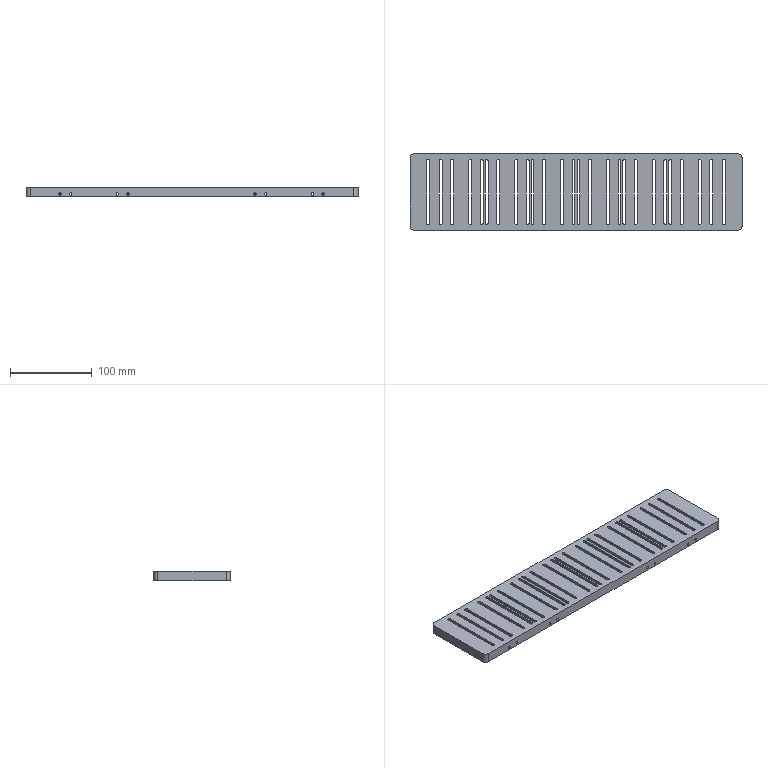Component | SolidWorks | MGL-PACK-02-00WeldedPlate2Assembly-1_MGL-PACK-02-01WeldedPlate2-1 | 1 solid | 295 faces | box 405 x 93 x 12 mm | volume 207669 mm3 | plane 151 | cylinder 92 | cone 52 | commonest cylinder face diameters 3.5 x48 3 x32 10 x8 4 x4
build123d program:
from build123d import *

# Parameters (mm, degrees)
SKETCH1_W             = 405
SKETCH1_H             = 93
BOSS_EXTRUDE1_DEPTH   = 12
CUT_EXTRUDE6_DEPTH    = 12
CUT_EXTRUDE1_DEPTH    = 12
LPATTERN1_COUNT       = 5
LPATTERN1_PITCH       = 56
CUT_EXTRUDE7_DEPTH    = 12
CUT_EXTRUDE2_DEPTH    = 6
FILLET1_R             = 5
M3_TAPPED_HOLE1_D     = 3
M3_TAPPED_HOLE1_DEPTH = 100
M3_TAPPED_HOLE1_TIP   = 0.9013
SKETCH10_W            = 9
SKETCH10_H            = 8
CUT_EXTRUDE5_DEPTH    = 2
CHAMFER2_SIZE         = 1
CHAMFER4_SIZE         = 1
CHAMFER4_SIZE2        = 3.732


with BuildPart() as part:
    # Sketch1 → Boss-Extrude1 (new body)
    with BuildSketch(Plane.XY):
        Rectangle(SKETCH1_W, SKETCH1_H)
    extrude(amount=BOSS_EXTRUDE1_DEPTH)

    # Sketch11 → Cut-Extrude6 (cut)
    with BuildSketch(Plane.XY.offset(12)):
        with BuildLine():
            Line((-178.75, 38), (-178.75, -38))
            ThreePointArc((-178.75, -38), (-180.5, -39.75), (-182.25, -38))
            Line((-182.25, -38), (-182.25, 38))
            ThreePointArc((-182.25, 38), (-180.5, 39.75), (-178.75, 38))
        make_face()
        with BuildLine():
            Line((182.25, 38), (182.25, -38))
            ThreePointArc((182.25, -38), (180.5, -39.75), (178.75, -38))
            Line((178.75, -38), (178.75, 38))
            ThreePointArc((178.75, 38), (180.5, 39.75), (182.25, 38))
        make_face()
        with BuildLine():
            Line((-163.25, 38), (-163.25, -38))
            ThreePointArc((-163.25, -38), (-165, -39.75), (-166.75, -38))
            Line((-166.75, -38), (-166.75, 38))
            ThreePointArc((-166.75, 38), (-165, 39.75), (-163.25, 38))
        make_face()
        with BuildLine():
            Line((166.75, 38), (166.75, -38))
            ThreePointArc((166.75, -38), (165, -39.75), (163.25, -38))
            Line((163.25, -38), (163.25, 38))
            ThreePointArc((163.25, 38), (165, 39.75), (166.75, 38))
        make_face()
    extrude(amount=-CUT_EXTRUDE6_DEPTH, mode=Mode.SUBTRACT)

    # Sketch2 → Cut-Extrude1 (cut)
    with BuildSketch(Plane.XY.offset(12)):
        with BuildLine():
            Line((-149.25, 38), (-149.25, -38))
            ThreePointArc((-149.25, -38), (-151, -39.75), (-152.75, -38))
            Line((-152.75, -38), (-152.75, 38))
            ThreePointArc((-152.75, 38), (-151, 39.75), (-149.25, 38))
        make_face()
        with BuildLine():
            Line((-127.25, 38), (-127.25, -38))
            ThreePointArc((-127.25, -38), (-129, -39.75), (-130.75, -38))
            Line((-130.75, -38), (-130.75, 38))
            ThreePointArc((-130.75, 38), (-129, 39.75), (-127.25, 38))
        make_face()
        with BuildLine():
            Line((-113.25, 38), (-113.25, -38))
            ThreePointArc((-113.25, -38), (-115, -39.75), (-116.75, -38))
            Line((-116.75, -38), (-116.75, 38))
            ThreePointArc((-116.75, 38), (-115, 39.75), (-113.25, 38))
        make_face()
        with BuildLine():
            Line((-107.25, 38), (-107.25, -38))
            ThreePointArc((-107.25, -38), (-109, -39.75), (-110.75, -38))
            Line((-110.75, -38), (-110.75, 38))
            ThreePointArc((-110.75, 38), (-109, 39.75), (-107.25, 38))
        make_face()
    cut_extrude1 = extrude(amount=-CUT_EXTRUDE1_DEPTH, mode=Mode.SUBTRACT)

    # LPattern1: Cut-Extrude1 ×5
    with Locations(*[(i * LPATTERN1_PITCH, 0, 0) for i in range(1, LPATTERN1_COUNT)]):
        add(cut_extrude1, mode=Mode.SUBTRACT)

    # Sketch12 → Cut-Extrude7 (cut)
    with BuildSketch(Plane.XY.offset(12)):
        with BuildLine():
            Line((131, 38), (131, -38))
            ThreePointArc((131, -38), (129, -40), (127, -38))
            Line((127, -38), (127, 38))
            ThreePointArc((127, 38), (129, 40), (131, 38))
        make_face()
        with BuildLine():
            Line((153, 38), (153, -38))
            ThreePointArc((153, -38), (151, -40), (149, -38))
            Line((149, -38), (149, 38))
            ThreePointArc((149, 38), (151, 40), (153, 38))
        make_face()
    extrude(amount=-CUT_EXTRUDE7_DEPTH, mode=Mode.SUBTRACT)

    # Sketch3 → Cut-Extrude2 (cut)
    with BuildSketch(Plane.XY.offset(12)):
        with BuildLine():
            Line((-185, 42), (185, 42))
            ThreePointArc((185, 42), (188.536, 40.536), (190, 37))
            Line((190, 37), (190, -37))
            ThreePointArc((190, -37), (188.536, -40.536), (185, -42))
            Line((185, -42), (-185, -42))
            ThreePointArc((-185, -42), (-188.536, -40.536), (-190, -37))
            Line((-190, -37), (-190, 37))
            ThreePointArc((-190, 37), (-188.536, 40.536), (-185, 42))
        make_face()
    extrude(amount=-CUT_EXTRUDE2_DEPTH, mode=Mode.SUBTRACT)

    # Fillet1
    fillet1_edges = [part.edges().sort_by_distance(p)[0] for p in [
        (-202.5, 46.5, 6),
        (202.5, 46.5, 6),
        (202.5, -46.5, 6),
        (-202.5, -46.5, 6),
    ]]
    fillet(fillet1_edges, radius=FILLET1_R)

    # M3 Tapped Hole1
    with Locations(Plane(origin=(0, -46.5, 0), x_dir=(-1, 0, 0), z_dir=(0, -1, 0))):
        with Locations((-161.05, -8.5), (-148.05, -8.5), (159.95, -8.5), (146.95, -8.5), (-91.05, -8.5), (-78.05, -8.5), (89.95, -8.5), (76.95, -8.5)):
            Hole(M3_TAPPED_HOLE1_D / 2, depth=M3_TAPPED_HOLE1_DEPTH)
            with Locations((0, 0, -(M3_TAPPED_HOLE1_DEPTH + M3_TAPPED_HOLE1_TIP / 2))):  # 118° drill point
                Cone(0, M3_TAPPED_HOLE1_D / 2, M3_TAPPED_HOLE1_TIP, mode=Mode.SUBTRACT)

    # Sketch10 → Cut-Extrude5 (cut)
    with BuildSketch(Plane.XY.offset(12)):
        with Locations((196.25, 31)):
            Rectangle(SKETCH10_W, SKETCH10_H)
        with Locations((196.25, -31)):
            Rectangle(SKETCH10_W, SKETCH10_H)
        with Locations((-196.25, 31)):
            Rectangle(SKETCH10_W, SKETCH10_H)
        with Locations((-196.25, -31)):
            Rectangle(SKETCH10_W, SKETCH10_H)
    extrude(amount=-CUT_EXTRUDE5_DEPTH, mode=Mode.SUBTRACT)

    # Chamfer2
    chamfer2_edges = [part.edges().sort_by_distance(p)[0] for p in [
        (191.75, 31, 12),
        (196.25, 27, 12),
        (200.75, 31, 12),
        (196.25, 35, 12),
        (191.75, -31, 12),
        (196.25, -35, 12),
        (200.75, -31, 12),
        (196.25, -27, 12),
        (-200.75, 31, 12),
        (-196.25, 27, 12),
        (-191.75, 31, 12),
        (-196.25, 35, 12),
        (-200.75, -31, 12),
        (-196.25, -35, 12),
        (-191.75, -31, 12),
        (-196.25, -27, 12),
    ]]
    chamfer(chamfer2_edges, length=CHAMFER2_SIZE)

    # Chamfer4
    chamfer4_edges = [part.edges().sort_by_distance(p)[0] for p in [
        (149, 0, 6),
        (153, 0, 6),
        (151, 40, 6),
        (151, -40, 6),
        (131, 0, 6),
        (129, 40, 6),
        (127, 0, 6),
        (129, -40, 6),
        (115, 39.75, 6),
        (113.25, 0, 6),
        (115, -39.75, 6),
        (116.75, 0, 6),
        (73, 39.75, 6),
        (71.25, 0, 6),
        (73, -39.75, 6),
        (74.75, 0, 6),
        (95, 39.75, 6),
        (93.25, 0, 6),
        (95, -39.75, 6),
        (96.75, 0, 6),
        (109, 39.75, 6),
        (107.25, 0, 6),
        (109, -39.75, 6),
        (110.75, 0, 6),
        (59, 39.75, 6),
        (57.25, 0, 6),
        (59, -39.75, 6),
        (60.75, 0, 6),
        (17, 39.75, 6),
        (15.25, 0, 6),
        (17, -39.75, 6),
        (18.75, 0, 6),
        (39, 39.75, 6),
        (37.25, 0, 6),
        (39, -39.75, 6),
        (40.75, 0, 6),
        (53, 39.75, 6),
        (51.25, 0, 6),
        (53, -39.75, 6),
        (54.75, 0, 6),
        (3, 39.75, 6),
        (1.25, 0, 6),
        (3, -39.75, 6),
        (4.75, 0, 6),
        (-39, 39.75, 6),
        (-40.75, 0, 6),
        (-39, -39.75, 6),
        (-37.25, 0, 6),
        (-17, 39.75, 6),
        (-18.75, 0, 6),
        (-17, -39.75, 6),
        (-15.25, 0, 6),
        (-3, 39.75, 6),
        (-4.75, 0, 6),
        (-3, -39.75, 6),
        (-1.25, 0, 6),
        (-51.25, 0, 6),
        (-53, 39.75, 6),
        (-54.75, 0, 6),
        (-53, -39.75, 6),
        (-93.25, 0, 6),
        (-95, 39.75, 6),
        (-96.75, 0, 6),
        (-95, -39.75, 6),
        (-71.25, 0, 6),
        (-73, 39.75, 6),
        (-74.75, 0, 6),
        (-73, -39.75, 6),
        (-57.25, 0, 6),
        (-59, 39.75, 6),
        (-60.75, 0, 6),
        (-59, -39.75, 6),
        (-107.25, 0, 6),
        (-109, 39.75, 6),
        (-110.75, 0, 6),
        (-109, -39.75, 6),
        (-113.25, 0, 6),
        (-115, 39.75, 6),
        (-116.75, 0, 6),
        (-115, -39.75, 6),
        (-127.25, 0, 6),
        (-129, 39.75, 6),
        (-130.75, 0, 6),
        (-129, -39.75, 6),
        (-149.25, 0, 6),
        (-151, 39.75, 6),
        (-152.75, 0, 6),
        (-151, -39.75, 6),
        (166.75, 0, 6),
        (165, 39.75, 6),
        (163.25, 0, 6),
        (165, -39.75, 6),
        (-163.25, 0, 6),
        (-165, 39.75, 6),
        (-166.75, 0, 6),
        (-165, -39.75, 6),
        (182.25, 0, 6),
        (180.5, 39.75, 6),
        (178.75, 0, 6),
        (180.5, -39.75, 6),
        (-178.75, 0, 6),
        (-180.5, 39.75, 6),
        (-182.25, 0, 6),
        (-180.5, -39.75, 6),
    ]]
    chamfer4_side = [part.faces().sort_by_distance(p)[0] for p in [
        (-0.4651, 0, 6),
    ]]
    chamfer(chamfer4_edges, length=CHAMFER4_SIZE, length2=CHAMFER4_SIZE2, reference=chamfer4_side[0])


solid = part.part

# Placed as in the assembly
solid = solid.moved(Location((0, 0, -251.6), (-180, 0, 180)))